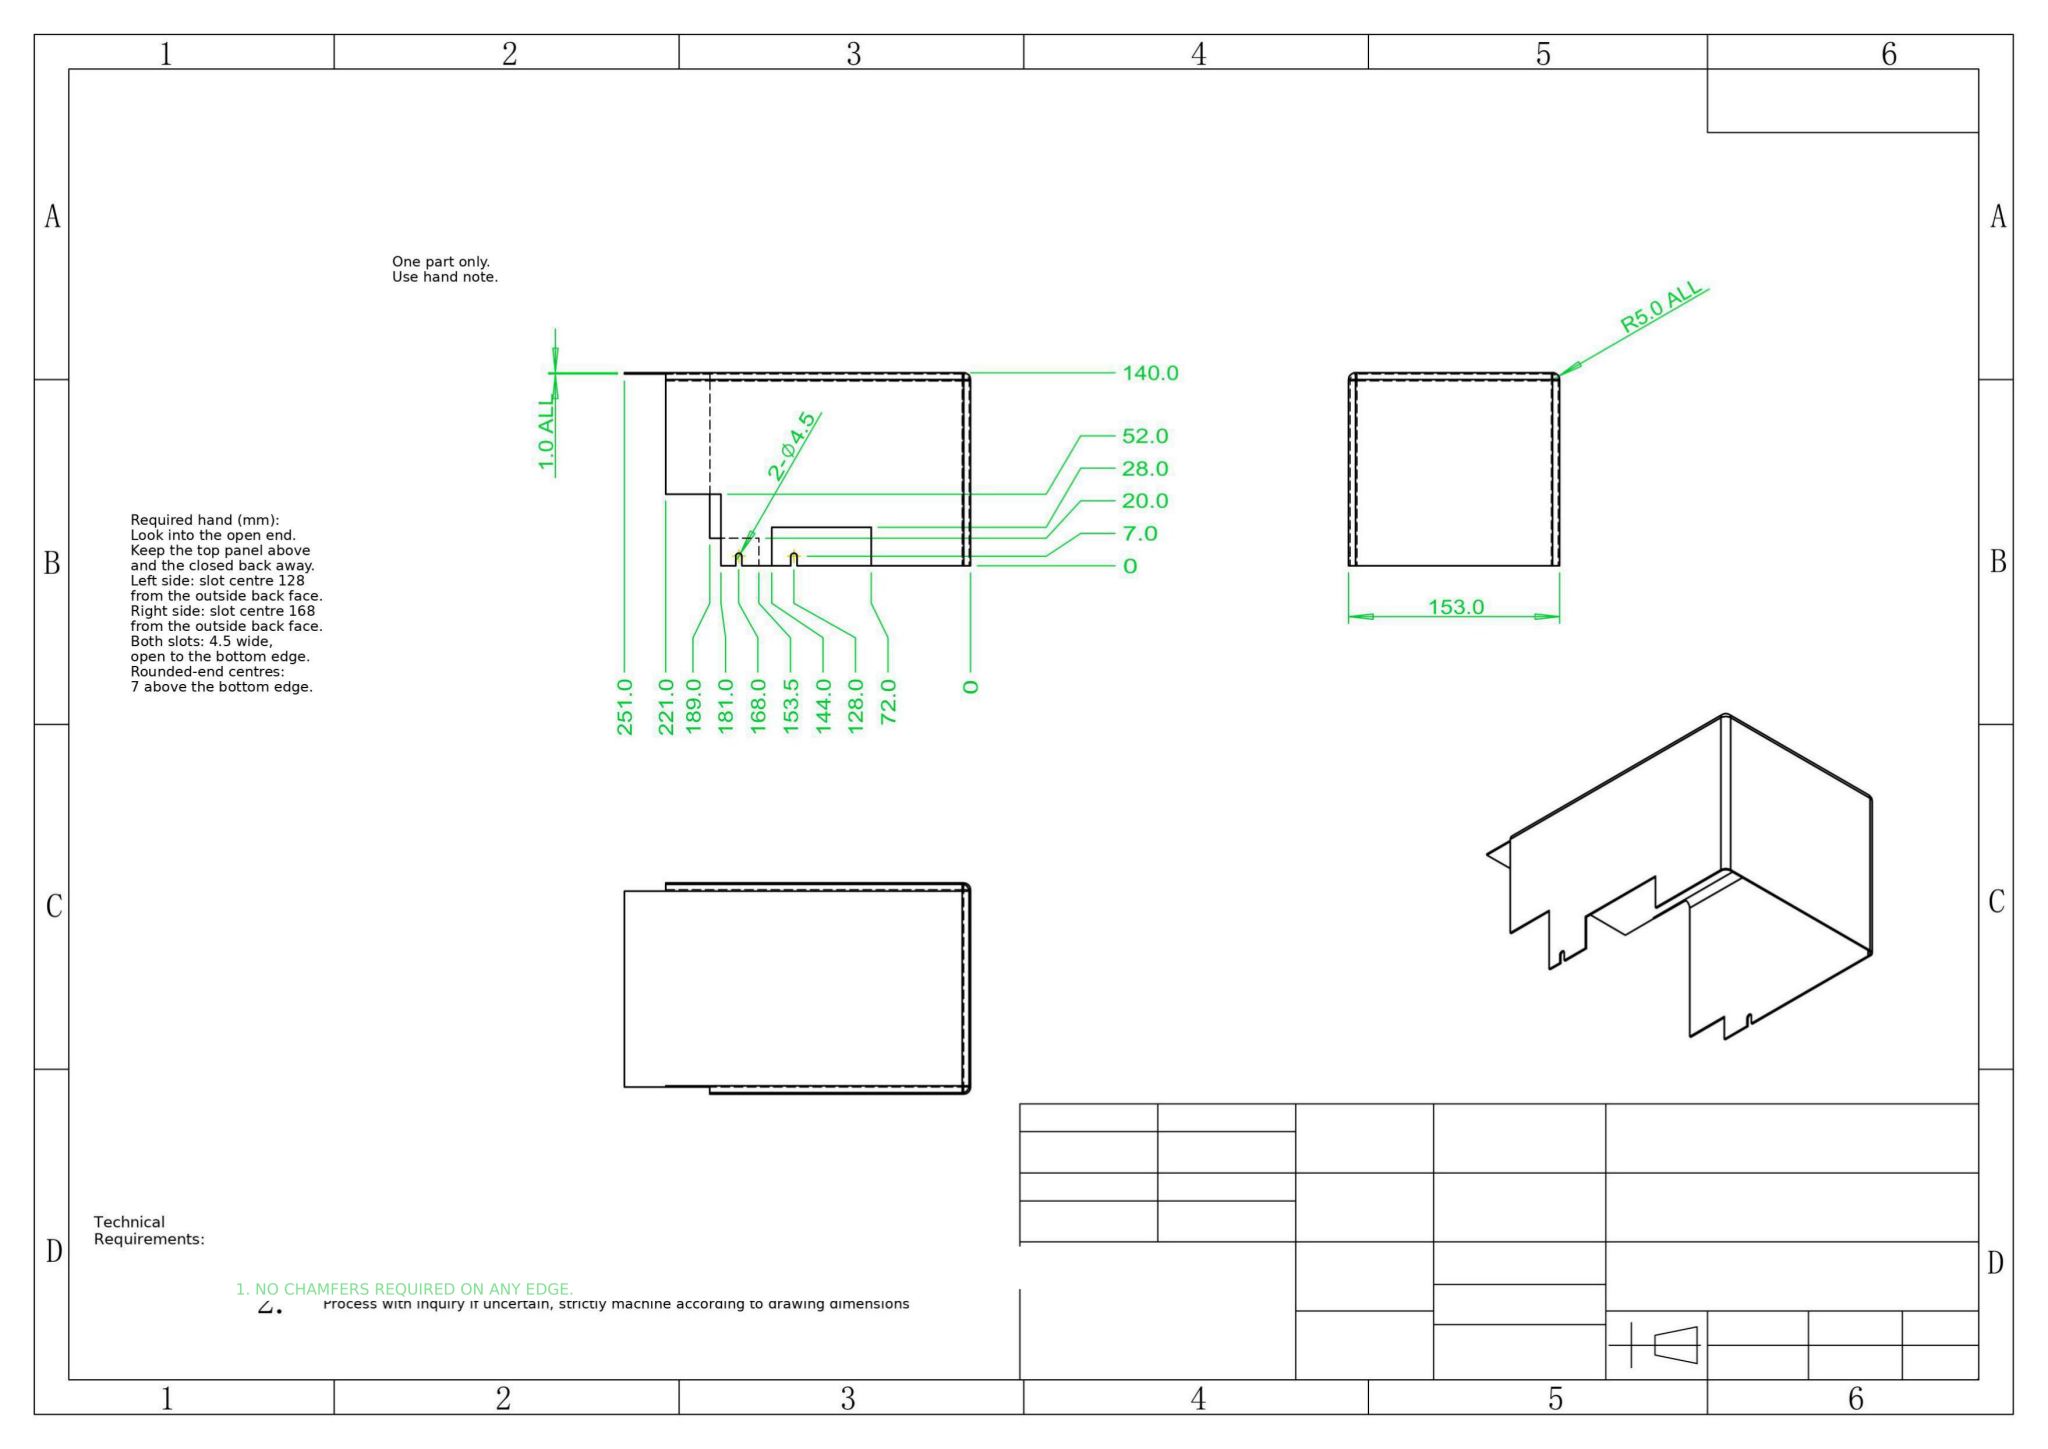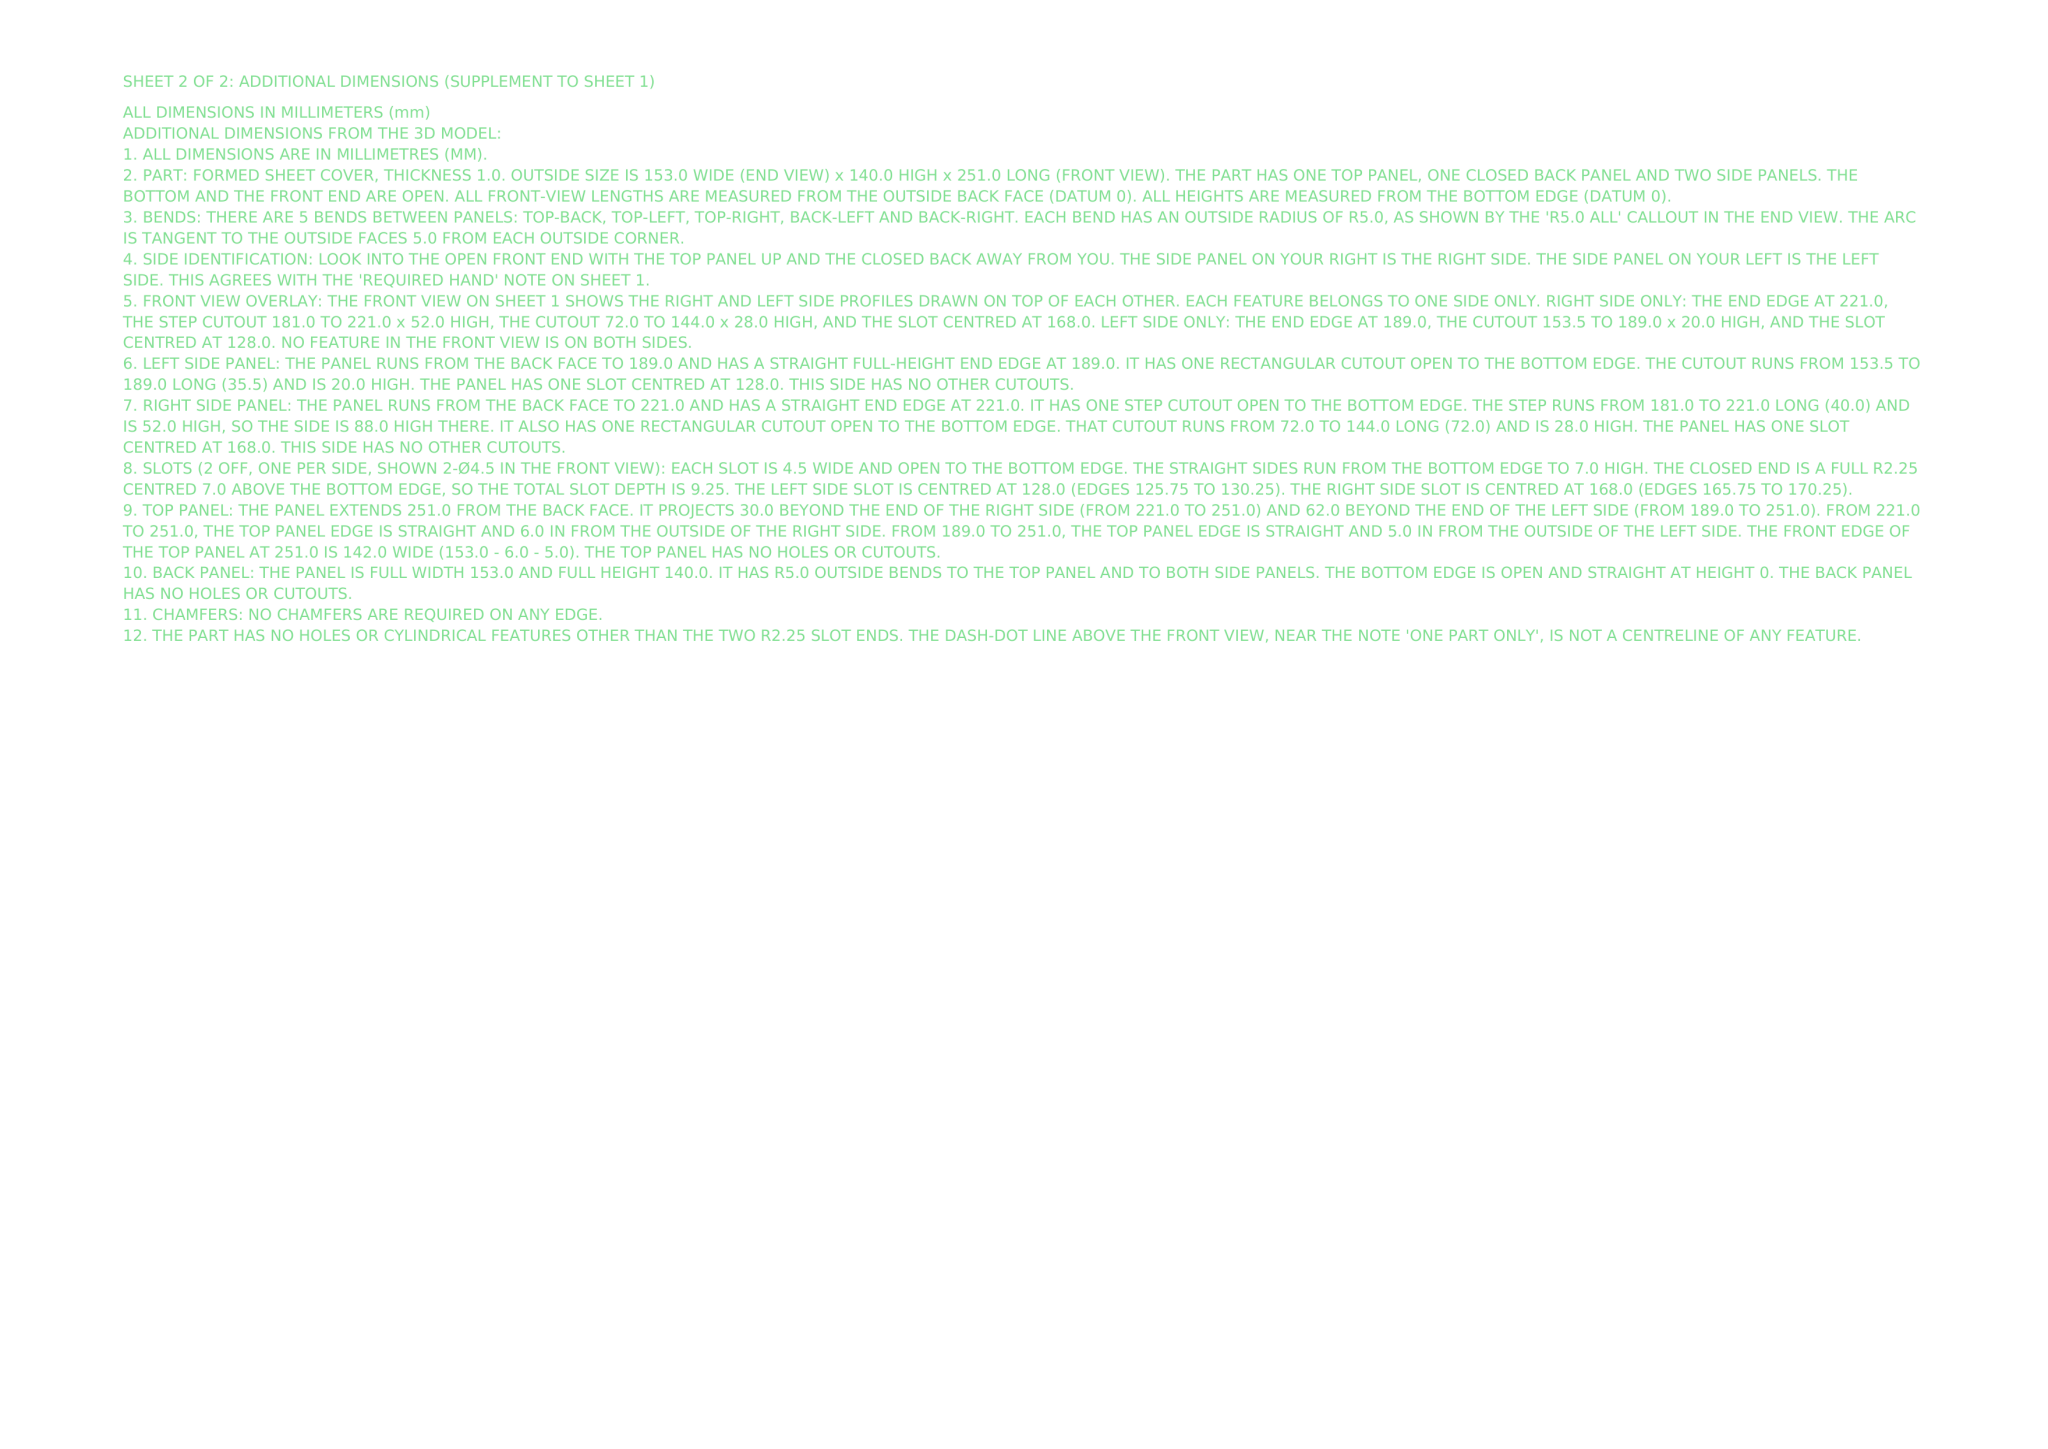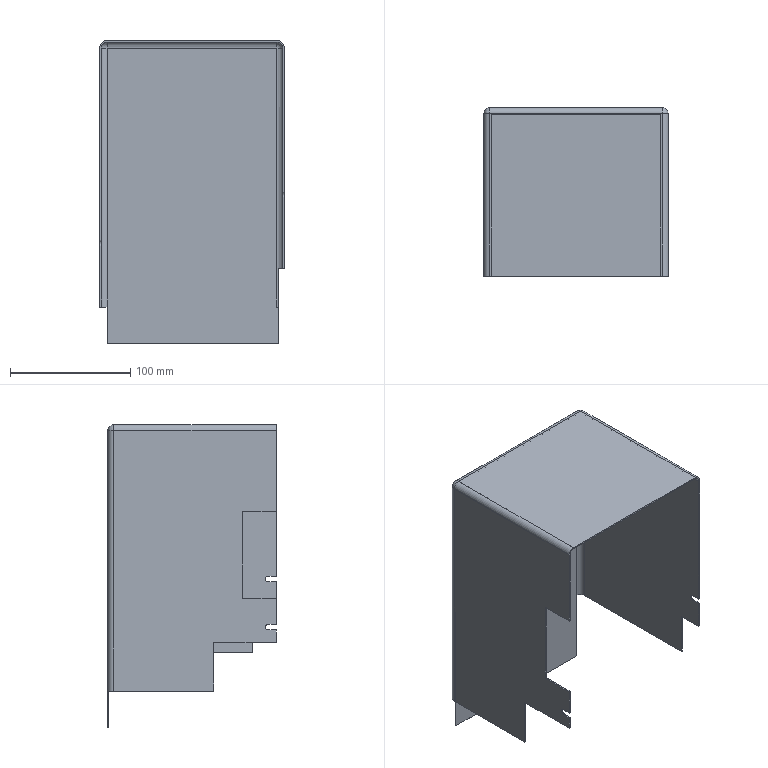Part | NX | mm | 1 solid | 45 faces | box 153 x 140 x 251 mm | volume 110976 mm3 | plane 29 | cylinder 12 | sphere 4 | commonest cylinder face diameters 10 x10 4.5 x2